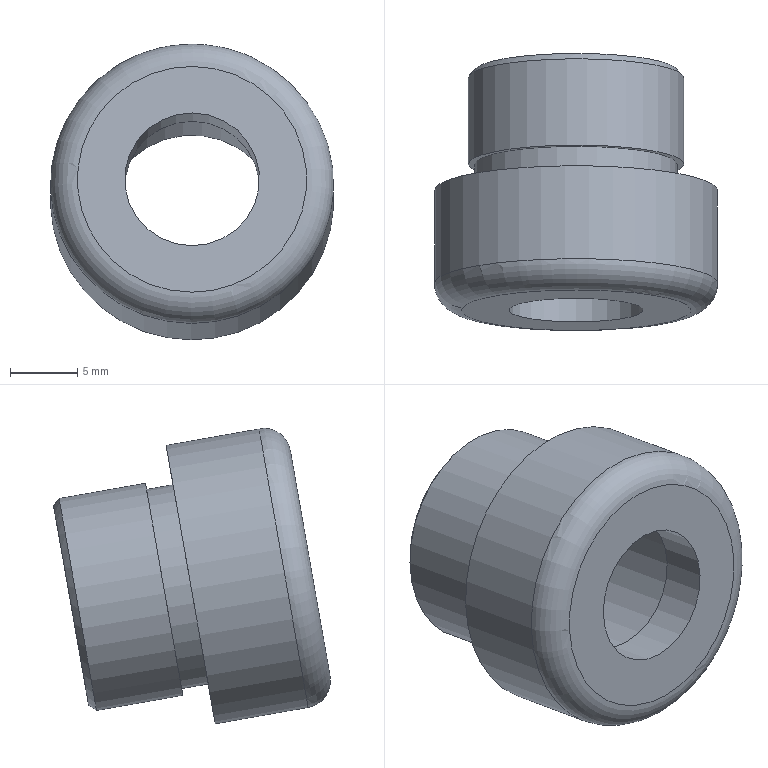Component | NX | SWING_ROD_BALL_JOINT_BASE | 1 solid | 12 faces | box 21 x 20.54 x 21.93 mm | volume 2618 mm3 | plane 5 | cylinder 5 | cone 1 | torus 1 | commonest cylinder face diameters 10 x1 13 x1 16 x1 15 x1 21 x1
STEP:
#1=CARTESIAN_POINT('',(0.,0.,0.));
#2=DIRECTION('',(0.,0.,1.));
#3=DIRECTION('',(1.,0.,0.));
#4=AXIS2_PLACEMENT_3D('',#1,#2,#3);
#5=CARTESIAN_POINT('',(84.128,207.703,139.261));
#6=VERTEX_POINT('',#5);
#7=CARTESIAN_POINT('',(84.166,208.571,144.184));
#8=DIRECTION('',(0.,-0.9848,0.1736));
#9=DIRECTION('',(-0.00764,-0.1736,-0.9848));
#10=AXIS2_PLACEMENT_3D('',#7,#8,#9);
#11=CIRCLE('',#10,5.);
#12=CARTESIAN_POINT('',(84.101,207.095,135.814));
#13=DIRECTION('',(0.,0.9848,-0.1736));
#14=DIRECTION('',(0.00764,0.1736,0.9848));
#15=AXIS2_PLACEMENT_3D('',#12,#13,#14);
#16=PLANE('',#15);
#17=CARTESIAN_POINT('',(3.5,-0.));
#18=CARTESIAN_POINT('',(3.5,8.66));
#19=CARTESIAN_POINT('',(11.,4.33));
#20=CARTESIAN_POINT('',(18.5,-0.));
#21=CARTESIAN_POINT('',(11.,-4.33));
#22=CARTESIAN_POINT('',(3.5,-8.66));
#23=CARTESIAN_POINT('',(3.5,-0.));
#24=(BOUNDED_CURVE()B_SPLINE_CURVE(2,(#17,#18,#19,#20,#21,#22,#23),.UNSPECIFIED.,.T.,.F.)B_SPLINE_CURVE_WITH_KNOTS((1,2,2,2,2,1),(-2.094,0.,2.094,4.189,6.283,8.378),.UNSPECIFIED.)CURVE()GEOMETRIC_REPRESENTATION_ITEM()RATIONAL_B_SPLINE_CURVE((1.,0.5,1.,0.5,1.,0.5,1.))REPRESENTATION_ITEM(''));
#25=(GEOMETRIC_REPRESENTATION_CONTEXT(2)PARAMETRIC_REPRESENTATION_CONTEXT()REPRESENTATION_CONTEXT('',''));
#26=DEFINITIONAL_REPRESENTATION('',(#24),#25);
#27=PCURVE('',#16,#26);
#28=CARTESIAN_POINT('',(84.166,226.298,141.059));
#29=DIRECTION('',(0.,-0.9848,0.1736));
#30=DIRECTION('',(-0.00764,-0.1736,-0.9848));
#31=AXIS2_PLACEMENT_3D('',#28,#29,#30);
#32=CYLINDRICAL_SURFACE('',#31,5.);
#33=CARTESIAN_POINT('',(0.,18.));
#34=DIRECTION('',(1.,0.));
#35=VECTOR('',#34,1.);
#36=LINE('',#33,#35);
#37=(GEOMETRIC_REPRESENTATION_CONTEXT(2)PARAMETRIC_REPRESENTATION_CONTEXT()REPRESENTATION_CONTEXT('',''));
#38=DEFINITIONAL_REPRESENTATION('',(#36),#37);
#39=PCURVE('',#32,#38);
#40=SURFACE_CURVE('',#11,(#27,#39),.PCURVE_S1.);
#41=EDGE_CURVE('',#6,#6,#40,.T.);
#42=ORIENTED_EDGE('',*,*,#41,.F.);
#43=EDGE_LOOP('',(#42));
#44=FACE_BOUND('',#43,.T.);
#45=CARTESIAN_POINT('',(84.101,207.095,135.814));
#46=VERTEX_POINT('',#45);
#47=CARTESIAN_POINT('',(84.166,208.571,144.184));
#48=DIRECTION('',(0.,-0.9848,0.1736));
#49=DIRECTION('',(-0.00764,-0.1736,-0.9848));
#50=AXIS2_PLACEMENT_3D('',#47,#48,#49);
#51=CIRCLE('',#50,8.5);
#52=CARTESIAN_POINT('',(0.,-0.));
#53=CARTESIAN_POINT('',(0.,14.722));
#54=CARTESIAN_POINT('',(12.75,7.361));
#55=CARTESIAN_POINT('',(25.5,-0.));
#56=CARTESIAN_POINT('',(12.75,-7.361));
#57=CARTESIAN_POINT('',(0.,-14.722));
#58=CARTESIAN_POINT('',(0.,-0.));
#59=(BOUNDED_CURVE()B_SPLINE_CURVE(2,(#52,#53,#54,#55,#56,#57,#58),.UNSPECIFIED.,.T.,.F.)B_SPLINE_CURVE_WITH_KNOTS((1,2,2,2,2,1),(-2.094,0.,2.094,4.189,6.283,8.378),.UNSPECIFIED.)CURVE()GEOMETRIC_REPRESENTATION_ITEM()RATIONAL_B_SPLINE_CURVE((1.,0.5,1.,0.5,1.,0.5,1.))REPRESENTATION_ITEM(''));
#60=(GEOMETRIC_REPRESENTATION_CONTEXT(2)PARAMETRIC_REPRESENTATION_CONTEXT()REPRESENTATION_CONTEXT('',''));
#61=DEFINITIONAL_REPRESENTATION('',(#59),#60);
#62=PCURVE('',#16,#61);
#63=CARTESIAN_POINT('',(84.166,210.541,143.837));
#64=DIRECTION('',(0.,-0.9848,0.1736));
#65=DIRECTION('',(-0.00764,-0.1736,-0.9848));
#66=AXIS2_PLACEMENT_3D('',#63,#64,#65);
#67=TOROIDAL_SURFACE('',#66,8.5,2.);
#68=CARTESIAN_POINT('',(0.,7.854));
#69=DIRECTION('',(1.,0.));
#70=VECTOR('',#69,1.);
#71=LINE('',#68,#70);
#72=(GEOMETRIC_REPRESENTATION_CONTEXT(2)PARAMETRIC_REPRESENTATION_CONTEXT()REPRESENTATION_CONTEXT('',''));
#73=DEFINITIONAL_REPRESENTATION('',(#71),#72);
#74=PCURVE('',#67,#73);
#75=SURFACE_CURVE('',#51,(#62,#74),.PCURVE_S1.);
#76=EDGE_CURVE('',#46,#46,#75,.T.);
#77=ORIENTED_EDGE('',*,*,#76,.T.);
#78=EDGE_LOOP('',(#77));
#79=FACE_BOUND('',#78,.T.);
#80=ADVANCED_FACE('',(#44,#79),#16,.F.);
#81=CARTESIAN_POINT('',(84.128,211.15,138.653));
#82=VERTEX_POINT('',#81);
#83=CARTESIAN_POINT('',(84.166,212.018,143.577));
#84=DIRECTION('',(0.,-0.9848,0.1736));
#85=DIRECTION('',(-0.00764,-0.1736,-0.9848));
#86=AXIS2_PLACEMENT_3D('',#83,#84,#85);
#87=CIRCLE('',#86,5.);
#88=CARTESIAN_POINT('',(0.,14.5));
#89=DIRECTION('',(1.,0.));
#90=VECTOR('',#89,1.);
#91=LINE('',#88,#90);
#92=(GEOMETRIC_REPRESENTATION_CONTEXT(2)PARAMETRIC_REPRESENTATION_CONTEXT()REPRESENTATION_CONTEXT('',''));
#93=DEFINITIONAL_REPRESENTATION('',(#91),#92);
#94=PCURVE('',#32,#93);
#95=CARTESIAN_POINT('',(84.128,211.15,138.653));
#96=DIRECTION('',(0.,-0.9848,0.1736));
#97=DIRECTION('',(-0.00764,-0.1736,-0.9848));
#98=AXIS2_PLACEMENT_3D('',#95,#96,#97);
#99=PLANE('',#98);
#100=CARTESIAN_POINT('',(-5.,-0.));
#101=DIRECTION('',(1.,0.));
#102=AXIS2_PLACEMENT_2D('',#100,#101);
#103=CIRCLE('',#102,5.);
#104=(GEOMETRIC_REPRESENTATION_CONTEXT(2)PARAMETRIC_REPRESENTATION_CONTEXT()REPRESENTATION_CONTEXT('',''));
#105=DEFINITIONAL_REPRESENTATION('',(#103),#104);
#106=PCURVE('',#99,#105);
#107=SURFACE_CURVE('',#87,(#94,#106),.PCURVE_S1.);
#108=EDGE_CURVE('',#82,#82,#107,.T.);
#109=ORIENTED_EDGE('',*,*,#108,.T.);
#110=CARTESIAN_POINT('',(84.128,211.15,138.653));
#111=CARTESIAN_POINT('',(84.128,207.703,139.261));
#112=B_SPLINE_CURVE_WITH_KNOTS('',1,(#110,#111),.UNSPECIFIED.,.F.,.F.,(2,2),(14.5,18.),.PIECEWISE_BEZIER_KNOTS.);
#113=CARTESIAN_POINT('',(6.283,0.));
#114=DIRECTION('',(0.,1.));
#115=VECTOR('',#114,1.);
#116=LINE('',#113,#115);
#117=(GEOMETRIC_REPRESENTATION_CONTEXT(2)PARAMETRIC_REPRESENTATION_CONTEXT()REPRESENTATION_CONTEXT('',''));
#118=DEFINITIONAL_REPRESENTATION('',(#116),#117);
#119=PCURVE('',#32,#118);
#120=CARTESIAN_POINT('',(0.,0.));
#121=DIRECTION('',(0.,1.));
#122=VECTOR('',#121,1.);
#123=LINE('',#120,#122);
#124=(GEOMETRIC_REPRESENTATION_CONTEXT(2)PARAMETRIC_REPRESENTATION_CONTEXT()REPRESENTATION_CONTEXT('',''));
#125=DEFINITIONAL_REPRESENTATION('',(#123),#124);
#126=PCURVE('',#32,#125);
#127=SEAM_CURVE('',#112,(#119,#126),.PCURVE_S1.);
#128=EDGE_CURVE('',#82,#6,#127,.T.);
#129=ORIENTED_EDGE('',*,*,#128,.T.);
#130=ORIENTED_EDGE('',*,*,#41,.F.);
#131=ORIENTED_EDGE('',*,*,#128,.F.);
#132=EDGE_LOOP('',(#109,#129,#130,#131));
#133=FACE_BOUND('',#132,.F.);
#134=ADVANCED_FACE('',(#133),#32,.F.);
#135=CARTESIAN_POINT('',(84.117,210.889,137.176));
#136=VERTEX_POINT('',#135);
#137=CARTESIAN_POINT('',(84.166,212.018,143.577));
#138=DIRECTION('',(0.,-0.9848,0.1736));
#139=DIRECTION('',(-0.00764,-0.1736,-0.9848));
#140=AXIS2_PLACEMENT_3D('',#137,#138,#139);
#141=CIRCLE('',#140,6.5);
#142=CARTESIAN_POINT('',(-5.,-0.));
#143=DIRECTION('',(1.,-0.));
#144=AXIS2_PLACEMENT_2D('',#142,#143);
#145=CIRCLE('',#144,6.5);
#146=(GEOMETRIC_REPRESENTATION_CONTEXT(2)PARAMETRIC_REPRESENTATION_CONTEXT()REPRESENTATION_CONTEXT('',''));
#147=DEFINITIONAL_REPRESENTATION('',(#145),#146);
#148=PCURVE('',#99,#147);
#149=CARTESIAN_POINT('',(84.166,226.298,141.059));
#150=DIRECTION('',(0.,-0.9848,0.1736));
#151=DIRECTION('',(-0.00764,-0.1736,-0.9848));
#152=AXIS2_PLACEMENT_3D('',#149,#150,#151);
#153=CYLINDRICAL_SURFACE('',#152,6.5);
#154=CARTESIAN_POINT('',(0.,14.5));
#155=DIRECTION('',(1.,0.));
#156=VECTOR('',#155,1.);
#157=LINE('',#154,#156);
#158=(GEOMETRIC_REPRESENTATION_CONTEXT(2)PARAMETRIC_REPRESENTATION_CONTEXT()REPRESENTATION_CONTEXT('',''));
#159=DEFINITIONAL_REPRESENTATION('',(#157),#158);
#160=PCURVE('',#153,#159);
#161=SURFACE_CURVE('',#141,(#148,#160),.PCURVE_S1.);
#162=EDGE_CURVE('',#136,#136,#161,.T.);
#163=ORIENTED_EDGE('',*,*,#162,.F.);
#164=EDGE_LOOP('',(#163));
#165=FACE_BOUND('',#164,.T.);
#166=ORIENTED_EDGE('',*,*,#108,.T.);
#167=EDGE_LOOP('',(#166));
#168=FACE_BOUND('',#167,.T.);
#169=ADVANCED_FACE('',(#165,#168),#99,.F.);
#170=CARTESIAN_POINT('',(84.117,225.169,134.658));
#171=VERTEX_POINT('',#170);
#172=CARTESIAN_POINT('',(84.166,226.298,141.059));
#173=DIRECTION('',(0.,-0.9848,0.1736));
#174=DIRECTION('',(-0.00764,-0.1736,-0.9848));
#175=AXIS2_PLACEMENT_3D('',#172,#173,#174);
#176=CIRCLE('',#175,6.5);
#177=CARTESIAN_POINT('',(0.,0.));
#178=DIRECTION('',(1.,0.));
#179=VECTOR('',#178,1.);
#180=LINE('',#177,#179);
#181=(GEOMETRIC_REPRESENTATION_CONTEXT(2)PARAMETRIC_REPRESENTATION_CONTEXT()REPRESENTATION_CONTEXT('',''));
#182=DEFINITIONAL_REPRESENTATION('',(#180),#181);
#183=PCURVE('',#153,#182);
#184=CARTESIAN_POINT('',(84.117,225.169,134.658));
#185=DIRECTION('',(0.,-0.9848,0.1736));
#186=DIRECTION('',(-0.00764,-0.1736,-0.9848));
#187=AXIS2_PLACEMENT_3D('',#184,#185,#186);
#188=PLANE('',#187);
#189=CARTESIAN_POINT('',(-6.5,-0.));
#190=DIRECTION('',(1.,-0.));
#191=AXIS2_PLACEMENT_2D('',#189,#190);
#192=CIRCLE('',#191,6.5);
#193=(GEOMETRIC_REPRESENTATION_CONTEXT(2)PARAMETRIC_REPRESENTATION_CONTEXT()REPRESENTATION_CONTEXT('',''));
#194=DEFINITIONAL_REPRESENTATION('',(#192),#193);
#195=PCURVE('',#188,#194);
#196=SURFACE_CURVE('',#176,(#183,#195),.PCURVE_S1.);
#197=EDGE_CURVE('',#171,#171,#196,.T.);
#198=ORIENTED_EDGE('',*,*,#197,.T.);
#199=CARTESIAN_POINT('',(84.117,225.169,134.658));
#200=CARTESIAN_POINT('',(84.117,210.889,137.176));
#201=B_SPLINE_CURVE_WITH_KNOTS('',1,(#199,#200),.UNSPECIFIED.,.F.,.F.,(2,2),(0.,14.5),.PIECEWISE_BEZIER_KNOTS.);
#202=CARTESIAN_POINT('',(6.283,0.));
#203=DIRECTION('',(0.,1.));
#204=VECTOR('',#203,1.);
#205=LINE('',#202,#204);
#206=(GEOMETRIC_REPRESENTATION_CONTEXT(2)PARAMETRIC_REPRESENTATION_CONTEXT()REPRESENTATION_CONTEXT('',''));
#207=DEFINITIONAL_REPRESENTATION('',(#205),#206);
#208=PCURVE('',#153,#207);
#209=CARTESIAN_POINT('',(0.,0.));
#210=DIRECTION('',(0.,1.));
#211=VECTOR('',#210,1.);
#212=LINE('',#209,#211);
#213=(GEOMETRIC_REPRESENTATION_CONTEXT(2)PARAMETRIC_REPRESENTATION_CONTEXT()REPRESENTATION_CONTEXT('',''));
#214=DEFINITIONAL_REPRESENTATION('',(#212),#213);
#215=PCURVE('',#153,#214);
#216=SEAM_CURVE('',#201,(#208,#215),.PCURVE_S1.);
#217=EDGE_CURVE('',#171,#136,#216,.T.);
#218=ORIENTED_EDGE('',*,*,#217,.T.);
#219=ORIENTED_EDGE('',*,*,#162,.F.);
#220=ORIENTED_EDGE('',*,*,#217,.F.);
#221=EDGE_LOOP('',(#198,#218,#219,#220));
#222=FACE_BOUND('',#221,.F.);
#223=ADVANCED_FACE('',(#222),#153,.F.);
#224=CARTESIAN_POINT('',(84.109,224.996,133.673));
#225=VERTEX_POINT('',#224);
#226=CARTESIAN_POINT('',(84.166,226.298,141.059));
#227=DIRECTION('',(0.,-0.9848,0.1736));
#228=DIRECTION('',(-0.00764,-0.1736,-0.9848));
#229=AXIS2_PLACEMENT_3D('',#226,#227,#228);
#230=CIRCLE('',#229,7.5);
#231=CARTESIAN_POINT('',(-6.5,-0.));
#232=DIRECTION('',(1.,0.));
#233=AXIS2_PLACEMENT_2D('',#231,#232);
#234=CIRCLE('',#233,7.5);
#235=(GEOMETRIC_REPRESENTATION_CONTEXT(2)PARAMETRIC_REPRESENTATION_CONTEXT()REPRESENTATION_CONTEXT('',''));
#236=DEFINITIONAL_REPRESENTATION('',(#234),#235);
#237=PCURVE('',#188,#236);
#238=CARTESIAN_POINT('',(84.166,226.298,141.059));
#239=DIRECTION('',(0.,-0.9848,0.1736));
#240=DIRECTION('',(-0.00764,-0.1736,-0.9848));
#241=AXIS2_PLACEMENT_3D('',#238,#239,#240);
#242=CONICAL_SURFACE('',#241,7.5,0.7854);
#243=CARTESIAN_POINT('',(0.,-0.));
#244=DIRECTION('',(1.,0.));
#245=VECTOR('',#244,1.);
#246=LINE('',#243,#245);
#247=(GEOMETRIC_REPRESENTATION_CONTEXT(2)PARAMETRIC_REPRESENTATION_CONTEXT()REPRESENTATION_CONTEXT('',''));
#248=DEFINITIONAL_REPRESENTATION('',(#246),#247);
#249=PCURVE('',#242,#248);
#250=SURFACE_CURVE('',#230,(#237,#249),.PCURVE_S1.);
#251=EDGE_CURVE('',#225,#225,#250,.T.);
#252=ORIENTED_EDGE('',*,*,#251,.F.);
#253=EDGE_LOOP('',(#252));
#254=FACE_BOUND('',#253,.T.);
#255=ORIENTED_EDGE('',*,*,#197,.T.);
#256=EDGE_LOOP('',(#255));
#257=FACE_BOUND('',#256,.T.);
#258=ADVANCED_FACE('',(#254,#257),#188,.F.);
#259=CARTESIAN_POINT('',(84.105,224.416,133.267));
#260=VERTEX_POINT('',#259);
#261=CARTESIAN_POINT('',(84.166,225.805,141.146));
#262=DIRECTION('',(0.,-0.9848,0.1736));
#263=DIRECTION('',(-0.00764,-0.1736,-0.9848));
#264=AXIS2_PLACEMENT_3D('',#261,#262,#263);
#265=CIRCLE('',#264,8.);
#266=CARTESIAN_POINT('',(0.,0.5));
#267=DIRECTION('',(1.,0.));
#268=VECTOR('',#267,1.);
#269=LINE('',#266,#268);
#270=(GEOMETRIC_REPRESENTATION_CONTEXT(2)PARAMETRIC_REPRESENTATION_CONTEXT()REPRESENTATION_CONTEXT('',''));
#271=DEFINITIONAL_REPRESENTATION('',(#269),#270);
#272=PCURVE('',#242,#271);
#273=CARTESIAN_POINT('',(84.166,226.298,141.059));
#274=DIRECTION('',(0.,-0.9848,0.1736));
#275=DIRECTION('',(-0.00764,-0.1736,-0.9848));
#276=AXIS2_PLACEMENT_3D('',#273,#274,#275);
#277=CYLINDRICAL_SURFACE('',#276,8.);
#278=CARTESIAN_POINT('',(0.,0.5));
#279=DIRECTION('',(1.,0.));
#280=VECTOR('',#279,1.);
#281=LINE('',#278,#280);
#282=(GEOMETRIC_REPRESENTATION_CONTEXT(2)PARAMETRIC_REPRESENTATION_CONTEXT()REPRESENTATION_CONTEXT('',''));
#283=DEFINITIONAL_REPRESENTATION('',(#281),#282);
#284=PCURVE('',#277,#283);
#285=SURFACE_CURVE('',#265,(#272,#284),.PCURVE_S1.);
#286=EDGE_CURVE('',#260,#260,#285,.T.);
#287=ORIENTED_EDGE('',*,*,#286,.F.);
#288=CARTESIAN_POINT('',(84.109,224.996,133.673));
#289=CARTESIAN_POINT('',(84.105,224.416,133.267));
#290=B_SPLINE_CURVE_WITH_KNOTS('',1,(#288,#289),.UNSPECIFIED.,.F.,.F.,(2,2),(-0.,0.7071),.PIECEWISE_BEZIER_KNOTS.);
#291=CARTESIAN_POINT('',(0.,0.));
#292=DIRECTION('',(0.,1.));
#293=VECTOR('',#292,1.);
#294=LINE('',#291,#293);
#295=(GEOMETRIC_REPRESENTATION_CONTEXT(2)PARAMETRIC_REPRESENTATION_CONTEXT()REPRESENTATION_CONTEXT('',''));
#296=DEFINITIONAL_REPRESENTATION('',(#294),#295);
#297=PCURVE('',#242,#296);
#298=CARTESIAN_POINT('',(6.283,0.));
#299=DIRECTION('',(0.,1.));
#300=VECTOR('',#299,1.);
#301=LINE('',#298,#300);
#302=(GEOMETRIC_REPRESENTATION_CONTEXT(2)PARAMETRIC_REPRESENTATION_CONTEXT()REPRESENTATION_CONTEXT('',''));
#303=DEFINITIONAL_REPRESENTATION('',(#301),#302);
#304=PCURVE('',#242,#303);
#305=SEAM_CURVE('',#290,(#297,#304),.PCURVE_S1.);
#306=EDGE_CURVE('',#225,#260,#305,.T.);
#307=ORIENTED_EDGE('',*,*,#306,.F.);
#308=ORIENTED_EDGE('',*,*,#251,.T.);
#309=ORIENTED_EDGE('',*,*,#306,.T.);
#310=EDGE_LOOP('',(#287,#307,#308,#309));
#311=FACE_BOUND('',#310,.T.);
#312=ADVANCED_FACE('',(#311),#242,.T.);
#313=CARTESIAN_POINT('',(84.105,218.015,134.396));
#314=VERTEX_POINT('',#313);
#315=CARTESIAN_POINT('',(84.166,219.404,142.274));
#316=DIRECTION('',(0.,-0.9848,0.1736));
#317=DIRECTION('',(-0.00764,-0.1736,-0.9848));
#318=AXIS2_PLACEMENT_3D('',#315,#316,#317);
#319=CIRCLE('',#318,8.);
#320=CARTESIAN_POINT('',(0.,7.));
#321=DIRECTION('',(1.,0.));
#322=VECTOR('',#321,1.);
#323=LINE('',#320,#322);
#324=(GEOMETRIC_REPRESENTATION_CONTEXT(2)PARAMETRIC_REPRESENTATION_CONTEXT()REPRESENTATION_CONTEXT('',''));
#325=DEFINITIONAL_REPRESENTATION('',(#323),#324);
#326=PCURVE('',#277,#325);
#327=CARTESIAN_POINT('',(84.105,218.015,134.396));
#328=DIRECTION('',(0.,0.9848,-0.1736));
#329=DIRECTION('',(0.00764,0.1736,0.9848));
#330=AXIS2_PLACEMENT_3D('',#327,#328,#329);
#331=PLANE('',#330);
#332=CARTESIAN_POINT('',(-0.,-0.));
#333=CARTESIAN_POINT('',(-0.,13.856));
#334=CARTESIAN_POINT('',(12.,6.928));
#335=CARTESIAN_POINT('',(24.,-0.));
#336=CARTESIAN_POINT('',(12.,-6.928));
#337=CARTESIAN_POINT('',(-0.,-13.856));
#338=CARTESIAN_POINT('',(-0.,-0.));
#339=(BOUNDED_CURVE()B_SPLINE_CURVE(2,(#332,#333,#334,#335,#336,#337,#338),.UNSPECIFIED.,.T.,.F.)B_SPLINE_CURVE_WITH_KNOTS((1,2,2,2,2,1),(-2.094,0.,2.094,4.189,6.283,8.378),.UNSPECIFIED.)CURVE()GEOMETRIC_REPRESENTATION_ITEM()RATIONAL_B_SPLINE_CURVE((1.,0.5,1.,0.5,1.,0.5,1.))REPRESENTATION_ITEM(''));
#340=(GEOMETRIC_REPRESENTATION_CONTEXT(2)PARAMETRIC_REPRESENTATION_CONTEXT()REPRESENTATION_CONTEXT('',''));
#341=DEFINITIONAL_REPRESENTATION('',(#339),#340);
#342=PCURVE('',#331,#341);
#343=SURFACE_CURVE('',#319,(#326,#342),.PCURVE_S1.);
#344=EDGE_CURVE('',#314,#314,#343,.T.);
#345=ORIENTED_EDGE('',*,*,#344,.F.);
#346=CARTESIAN_POINT('',(84.105,224.416,133.267));
#347=CARTESIAN_POINT('',(84.105,218.015,134.396));
#348=B_SPLINE_CURVE_WITH_KNOTS('',1,(#346,#347),.UNSPECIFIED.,.F.,.F.,(2,2),(0.5,7.),.PIECEWISE_BEZIER_KNOTS.);
#349=CARTESIAN_POINT('',(0.,0.));
#350=DIRECTION('',(0.,1.));
#351=VECTOR('',#350,1.);
#352=LINE('',#349,#351);
#353=(GEOMETRIC_REPRESENTATION_CONTEXT(2)PARAMETRIC_REPRESENTATION_CONTEXT()REPRESENTATION_CONTEXT('',''));
#354=DEFINITIONAL_REPRESENTATION('',(#352),#353);
#355=PCURVE('',#277,#354);
#356=CARTESIAN_POINT('',(6.283,0.));
#357=DIRECTION('',(0.,1.));
#358=VECTOR('',#357,1.);
#359=LINE('',#356,#358);
#360=(GEOMETRIC_REPRESENTATION_CONTEXT(2)PARAMETRIC_REPRESENTATION_CONTEXT()REPRESENTATION_CONTEXT('',''));
#361=DEFINITIONAL_REPRESENTATION('',(#359),#360);
#362=PCURVE('',#277,#361);
#363=SEAM_CURVE('',#348,(#355,#362),.PCURVE_S1.);
#364=EDGE_CURVE('',#260,#314,#363,.T.);
#365=ORIENTED_EDGE('',*,*,#364,.F.);
#366=ORIENTED_EDGE('',*,*,#286,.T.);
#367=ORIENTED_EDGE('',*,*,#364,.T.);
#368=EDGE_LOOP('',(#345,#365,#366,#367));
#369=FACE_BOUND('',#368,.T.);
#370=ADVANCED_FACE('',(#369),#277,.T.);
#371=CARTESIAN_POINT('',(84.109,218.102,134.888));
#372=VERTEX_POINT('',#371);
#373=CARTESIAN_POINT('',(84.166,219.404,142.274));
#374=DIRECTION('',(0.,-0.9848,0.1736));
#375=DIRECTION('',(-0.00764,-0.1736,-0.9848));
#376=AXIS2_PLACEMENT_3D('',#373,#374,#375);
#377=CIRCLE('',#376,7.5);
#378=CARTESIAN_POINT('',(0.5,-0.));
#379=CARTESIAN_POINT('',(0.5,12.99));
#380=CARTESIAN_POINT('',(11.75,6.495));
#381=CARTESIAN_POINT('',(23.,-0.));
#382=CARTESIAN_POINT('',(11.75,-6.495));
#383=CARTESIAN_POINT('',(0.5,-12.99));
#384=CARTESIAN_POINT('',(0.5,-0.));
#385=(BOUNDED_CURVE()B_SPLINE_CURVE(2,(#378,#379,#380,#381,#382,#383,#384),.UNSPECIFIED.,.T.,.F.)B_SPLINE_CURVE_WITH_KNOTS((1,2,2,2,2,1),(-2.094,0.,2.094,4.189,6.283,8.378),.UNSPECIFIED.)CURVE()GEOMETRIC_REPRESENTATION_ITEM()RATIONAL_B_SPLINE_CURVE((1.,0.5,1.,0.5,1.,0.5,1.))REPRESENTATION_ITEM(''));
#386=(GEOMETRIC_REPRESENTATION_CONTEXT(2)PARAMETRIC_REPRESENTATION_CONTEXT()REPRESENTATION_CONTEXT('',''));
#387=DEFINITIONAL_REPRESENTATION('',(#385),#386);
#388=PCURVE('',#331,#387);
#389=CARTESIAN_POINT('',(84.166,226.298,141.059));
#390=DIRECTION('',(0.,-0.9848,0.1736));
#391=DIRECTION('',(-0.00764,-0.1736,-0.9848));
#392=AXIS2_PLACEMENT_3D('',#389,#390,#391);
#393=CYLINDRICAL_SURFACE('',#392,7.5);
#394=CARTESIAN_POINT('',(0.,7.));
#395=DIRECTION('',(1.,0.));
#396=VECTOR('',#395,1.);
#397=LINE('',#394,#396);
#398=(GEOMETRIC_REPRESENTATION_CONTEXT(2)PARAMETRIC_REPRESENTATION_CONTEXT()REPRESENTATION_CONTEXT('',''));
#399=DEFINITIONAL_REPRESENTATION('',(#397),#398);
#400=PCURVE('',#393,#399);
#401=SURFACE_CURVE('',#377,(#388,#400),.PCURVE_S1.);
#402=EDGE_CURVE('',#372,#372,#401,.T.);
#403=ORIENTED_EDGE('',*,*,#402,.F.);
#404=EDGE_LOOP('',(#403));
#405=FACE_BOUND('',#404,.T.);
#406=ORIENTED_EDGE('',*,*,#344,.T.);
#407=EDGE_LOOP('',(#406));
#408=FACE_BOUND('',#407,.T.);
#409=ADVANCED_FACE('',(#405,#408),#331,.F.);
#410=CARTESIAN_POINT('',(84.109,216.132,135.236));
#411=VERTEX_POINT('',#410);
#412=CARTESIAN_POINT('',(84.166,217.435,142.622));
#413=DIRECTION('',(0.,-0.9848,0.1736));
#414=DIRECTION('',(-0.00764,-0.1736,-0.9848));
#415=AXIS2_PLACEMENT_3D('',#412,#413,#414);
#416=CIRCLE('',#415,7.5);
#417=CARTESIAN_POINT('',(0.,9.));
#418=DIRECTION('',(1.,0.));
#419=VECTOR('',#418,1.);
#420=LINE('',#417,#419);
#421=(GEOMETRIC_REPRESENTATION_CONTEXT(2)PARAMETRIC_REPRESENTATION_CONTEXT()REPRESENTATION_CONTEXT('',''));
#422=DEFINITIONAL_REPRESENTATION('',(#420),#421);
#423=PCURVE('',#393,#422);
#424=CARTESIAN_POINT('',(84.109,216.132,135.236));
#425=DIRECTION('',(0.,-0.9848,0.1736));
#426=DIRECTION('',(-0.00764,-0.1736,-0.9848));
#427=AXIS2_PLACEMENT_3D('',#424,#425,#426);
#428=PLANE('',#427);
#429=CARTESIAN_POINT('',(-7.5,-0.));
#430=DIRECTION('',(1.,0.));
#431=AXIS2_PLACEMENT_2D('',#429,#430);
#432=CIRCLE('',#431,7.5);
#433=(GEOMETRIC_REPRESENTATION_CONTEXT(2)PARAMETRIC_REPRESENTATION_CONTEXT()REPRESENTATION_CONTEXT('',''));
#434=DEFINITIONAL_REPRESENTATION('',(#432),#433);
#435=PCURVE('',#428,#434);
#436=SURFACE_CURVE('',#416,(#423,#435),.PCURVE_S1.);
#437=EDGE_CURVE('',#411,#411,#436,.T.);
#438=ORIENTED_EDGE('',*,*,#437,.F.);
#439=CARTESIAN_POINT('',(84.109,218.102,134.888));
#440=CARTESIAN_POINT('',(84.109,216.132,135.236));
#441=B_SPLINE_CURVE_WITH_KNOTS('',1,(#439,#440),.UNSPECIFIED.,.F.,.F.,(2,2),(7.,9.),.PIECEWISE_BEZIER_KNOTS.);
#442=CARTESIAN_POINT('',(0.,0.));
#443=DIRECTION('',(0.,1.));
#444=VECTOR('',#443,1.);
#445=LINE('',#442,#444);
#446=(GEOMETRIC_REPRESENTATION_CONTEXT(2)PARAMETRIC_REPRESENTATION_CONTEXT()REPRESENTATION_CONTEXT('',''));
#447=DEFINITIONAL_REPRESENTATION('',(#445),#446);
#448=PCURVE('',#393,#447);
#449=CARTESIAN_POINT('',(6.283,0.));
#450=DIRECTION('',(0.,1.));
#451=VECTOR('',#450,1.);
#452=LINE('',#449,#451);
#453=(GEOMETRIC_REPRESENTATION_CONTEXT(2)PARAMETRIC_REPRESENTATION_CONTEXT()REPRESENTATION_CONTEXT('',''));
#454=DEFINITIONAL_REPRESENTATION('',(#452),#453);
#455=PCURVE('',#393,#454);
#456=SEAM_CURVE('',#441,(#448,#455),.PCURVE_S1.);
#457=EDGE_CURVE('',#372,#411,#456,.T.);
#458=ORIENTED_EDGE('',*,*,#457,.F.);
#459=ORIENTED_EDGE('',*,*,#402,.T.);
#460=ORIENTED_EDGE('',*,*,#457,.T.);
#461=EDGE_LOOP('',(#438,#458,#459,#460));
#462=FACE_BOUND('',#461,.T.);
#463=ADVANCED_FACE('',(#462),#393,.T.);
#464=CARTESIAN_POINT('',(84.086,215.611,132.281));
#465=VERTEX_POINT('',#464);
#466=CARTESIAN_POINT('',(84.166,217.435,142.622));
#467=DIRECTION('',(0.,-0.9848,0.1736));
#468=DIRECTION('',(-0.00764,-0.1736,-0.9848));
#469=AXIS2_PLACEMENT_3D('',#466,#467,#468);
#470=CIRCLE('',#469,10.5);
#471=CARTESIAN_POINT('',(-7.5,-0.));
#472=DIRECTION('',(1.,0.));
#473=AXIS2_PLACEMENT_2D('',#471,#472);
#474=CIRCLE('',#473,10.5);
#475=(GEOMETRIC_REPRESENTATION_CONTEXT(2)PARAMETRIC_REPRESENTATION_CONTEXT()REPRESENTATION_CONTEXT('',''));
#476=DEFINITIONAL_REPRESENTATION('',(#474),#475);
#477=PCURVE('',#428,#476);
#478=CARTESIAN_POINT('',(84.166,226.298,141.059));
#479=DIRECTION('',(0.,-0.9848,0.1736));
#480=DIRECTION('',(-0.00764,-0.1736,-0.9848));
#481=AXIS2_PLACEMENT_3D('',#478,#479,#480);
#482=CYLINDRICAL_SURFACE('',#481,10.5);
#483=CARTESIAN_POINT('',(0.,9.));
#484=DIRECTION('',(1.,0.));
#485=VECTOR('',#484,1.);
#486=LINE('',#483,#485);
#487=(GEOMETRIC_REPRESENTATION_CONTEXT(2)PARAMETRIC_REPRESENTATION_CONTEXT()REPRESENTATION_CONTEXT('',''));
#488=DEFINITIONAL_REPRESENTATION('',(#486),#487);
#489=PCURVE('',#482,#488);
#490=SURFACE_CURVE('',#470,(#477,#489),.PCURVE_S1.);
#491=EDGE_CURVE('',#465,#465,#490,.T.);
#492=ORIENTED_EDGE('',*,*,#491,.F.);
#493=EDGE_LOOP('',(#492));
#494=FACE_BOUND('',#493,.T.);
#495=ORIENTED_EDGE('',*,*,#437,.T.);
#496=EDGE_LOOP('',(#495));
#497=FACE_BOUND('',#496,.T.);
#498=ADVANCED_FACE('',(#494,#497),#428,.F.);
#499=CARTESIAN_POINT('',(84.086,208.718,133.497));
#500=VERTEX_POINT('',#499);
#501=CARTESIAN_POINT('',(84.166,210.541,143.837));
#502=DIRECTION('',(0.,-0.9848,0.1736));
#503=DIRECTION('',(-0.00764,-0.1736,-0.9848));
#504=AXIS2_PLACEMENT_3D('',#501,#502,#503);
#505=CIRCLE('',#504,10.5);
#506=CARTESIAN_POINT('',(0.,16.));
#507=DIRECTION('',(1.,0.));
#508=VECTOR('',#507,1.);
#509=LINE('',#506,#508);
#510=(GEOMETRIC_REPRESENTATION_CONTEXT(2)PARAMETRIC_REPRESENTATION_CONTEXT()REPRESENTATION_CONTEXT('',''));
#511=DEFINITIONAL_REPRESENTATION('',(#509),#510);
#512=PCURVE('',#482,#511);
#513=CARTESIAN_POINT('',(0.,6.283));
#514=DIRECTION('',(1.,0.));
#515=VECTOR('',#514,1.);
#516=LINE('',#513,#515);
#517=(GEOMETRIC_REPRESENTATION_CONTEXT(2)PARAMETRIC_REPRESENTATION_CONTEXT()REPRESENTATION_CONTEXT('',''));
#518=DEFINITIONAL_REPRESENTATION('',(#516),#517);
#519=PCURVE('',#67,#518);
#520=SURFACE_CURVE('',#505,(#512,#519),.PCURVE_S1.);
#521=EDGE_CURVE('',#500,#500,#520,.T.);
#522=ORIENTED_EDGE('',*,*,#521,.F.);
#523=CARTESIAN_POINT('',(84.086,215.611,132.281));
#524=CARTESIAN_POINT('',(84.086,208.718,133.497));
#525=B_SPLINE_CURVE_WITH_KNOTS('',1,(#523,#524),.UNSPECIFIED.,.F.,.F.,(2,2),(9.,16.),.PIECEWISE_BEZIER_KNOTS.);
#526=CARTESIAN_POINT('',(0.,0.));
#527=DIRECTION('',(0.,1.));
#528=VECTOR('',#527,1.);
#529=LINE('',#526,#528);
#530=(GEOMETRIC_REPRESENTATION_CONTEXT(2)PARAMETRIC_REPRESENTATION_CONTEXT()REPRESENTATION_CONTEXT('',''));
#531=DEFINITIONAL_REPRESENTATION('',(#529),#530);
#532=PCURVE('',#482,#531);
#533=CARTESIAN_POINT('',(6.283,0.));
#534=DIRECTION('',(0.,1.));
#535=VECTOR('',#534,1.);
#536=LINE('',#533,#535);
#537=(GEOMETRIC_REPRESENTATION_CONTEXT(2)PARAMETRIC_REPRESENTATION_CONTEXT()REPRESENTATION_CONTEXT('',''));
#538=DEFINITIONAL_REPRESENTATION('',(#536),#537);
#539=PCURVE('',#482,#538);
#540=SEAM_CURVE('',#525,(#532,#539),.PCURVE_S1.);
#541=EDGE_CURVE('',#465,#500,#540,.T.);
#542=ORIENTED_EDGE('',*,*,#541,.F.);
#543=ORIENTED_EDGE('',*,*,#491,.T.);
#544=ORIENTED_EDGE('',*,*,#541,.T.);
#545=EDGE_LOOP('',(#522,#542,#543,#544));
#546=FACE_BOUND('',#545,.T.);
#547=ADVANCED_FACE('',(#546),#482,.T.);
#548=ORIENTED_EDGE('',*,*,#76,.F.);
#549=CARTESIAN_POINT('',(84.086,208.718,133.497));
#550=CARTESIAN_POINT('',(84.086,208.191,133.59));
#551=CARTESIAN_POINT('',(84.087,207.708,133.848));
#552=CARTESIAN_POINT('',(84.09,207.323,134.247));
#553=CARTESIAN_POINT('',(84.093,207.08,134.745));
#554=CARTESIAN_POINT('',(84.097,207.003,135.287));
#555=CARTESIAN_POINT('',(84.101,207.095,135.814));
#556=(BOUNDED_CURVE()B_SPLINE_CURVE(6,(#549,#550,#551,#552,#553,#554,#555),.UNSPECIFIED.,.F.,.F.)B_SPLINE_CURVE_WITH_KNOTS((7,7),(0.,1.571),.PIECEWISE_BEZIER_KNOTS.)CURVE()GEOMETRIC_REPRESENTATION_ITEM()RATIONAL_B_SPLINE_CURVE((1.031,1.01,0.9979,0.994,0.9979,1.01,1.031))REPRESENTATION_ITEM(''));
#557=CARTESIAN_POINT('',(0.,6.283));
#558=DIRECTION('',(0.,1.));
#559=VECTOR('',#558,1.);
#560=LINE('',#557,#559);
#561=(GEOMETRIC_REPRESENTATION_CONTEXT(2)PARAMETRIC_REPRESENTATION_CONTEXT()REPRESENTATION_CONTEXT('',''));
#562=DEFINITIONAL_REPRESENTATION('',(#560),#561);
#563=PCURVE('',#67,#562);
#564=CARTESIAN_POINT('',(6.283,6.283));
#565=DIRECTION('',(0.,1.));
#566=VECTOR('',#565,1.);
#567=LINE('',#564,#566);
#568=(GEOMETRIC_REPRESENTATION_CONTEXT(2)PARAMETRIC_REPRESENTATION_CONTEXT()REPRESENTATION_CONTEXT('',''));
#569=DEFINITIONAL_REPRESENTATION('',(#567),#568);
#570=PCURVE('',#67,#569);
#571=SEAM_CURVE('',#556,(#563,#570),.PCURVE_S1.);
#572=EDGE_CURVE('',#500,#46,#571,.T.);
#573=ORIENTED_EDGE('',*,*,#572,.F.);
#574=ORIENTED_EDGE('',*,*,#521,.T.);
#575=ORIENTED_EDGE('',*,*,#572,.T.);
#576=EDGE_LOOP('',(#548,#573,#574,#575));
#577=FACE_BOUND('',#576,.T.);
#578=ADVANCED_FACE('',(#577),#67,.T.);
#579=CLOSED_SHELL('',(#80,#134,#169,#223,#258,#312,#370,#409,#463,#498,#547,#578));
#580=MANIFOLD_SOLID_BREP('',#579);
#581=(LENGTH_UNIT()NAMED_UNIT(*)SI_UNIT(.MILLI.,.METRE.));
#582=UNCERTAINTY_MEASURE_WITH_UNIT(LENGTH_MEASURE(0.00001),#581,'','');
#583=(NAMED_UNIT(*)PLANE_ANGLE_UNIT()SI_UNIT($,.RADIAN.));
#584=(NAMED_UNIT(*)SI_UNIT($,.STERADIAN.)SOLID_ANGLE_UNIT());
#585=(GEOMETRIC_REPRESENTATION_CONTEXT(3)GLOBAL_UNCERTAINTY_ASSIGNED_CONTEXT((#582))GLOBAL_UNIT_ASSIGNED_CONTEXT((#581,#583,#584))REPRESENTATION_CONTEXT('',''));
#586=ADVANCED_BREP_SHAPE_REPRESENTATION('',(#4,#580),#585);